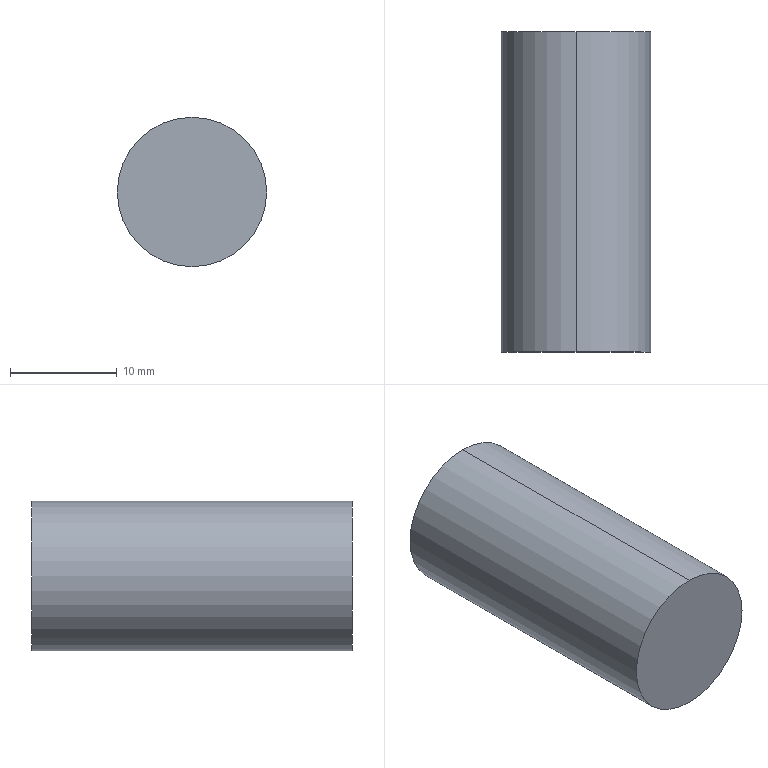Component | SolidWorks | DowelPin14X30-1 | 1 solid | 4 faces | box 14 x 30 x 14 mm | volume 4618 mm3 | cylinder 2 | plane 2 | commonest cylinder face diameters 14 x2
build123d program:
from build123d import *

# Parameters (mm, degrees)
SKETCH1_R           = 7
BOSS_EXTRUDE1_DEPTH = 30


with BuildPart() as part:
    # Sketch1 → Boss-Extrude1 (new body)
    with BuildSketch(Plane(origin=(0, 0, 0), x_dir=(1, 0, 0), z_dir=(0, 1, 0))):
        with Locations(Location((0, 0, 0), (0, 0, 270))):
            Circle(SKETCH1_R)
    extrude(amount=BOSS_EXTRUDE1_DEPTH)


solid = part.part

# Placed as in the assembly
solid = solid.moved(Location((-70.619, 73.047, -52), (0, 0, 0)))
STEP:
#1=COLOUR_RGB('',0.7922,0.8196,0.9333);
#2=FILL_AREA_STYLE_COLOUR('',#1);
#3=FILL_AREA_STYLE('',(#2));
#4=SURFACE_STYLE_FILL_AREA(#3);
#5=SURFACE_SIDE_STYLE('',(#4));
#6=SURFACE_STYLE_USAGE(.BOTH.,#5);
#7=PRESENTATION_STYLE_ASSIGNMENT((#6));
#8=CARTESIAN_POINT('',(-2.78,4.057,-1.772));
#9=VERTEX_POINT('',#8);
#10=CARTESIAN_POINT('',(-2.78,4.057,-2.323));
#11=VERTEX_POINT('',#10);
#12=CARTESIAN_POINT('',(-2.78,4.057,-2.047));
#13=DIRECTION('',(0.,1.,0.));
#14=DIRECTION('',(0.,0.,1.));
#15=AXIS2_PLACEMENT_3D('',#12,#13,#14);
#16=CIRCLE('',#15,0.2756);
#17=EDGE_CURVE('',#9,#11,#16,.T.);
#18=ORIENTED_EDGE('',*,*,#17,.F.);
#19=CARTESIAN_POINT('',(-2.78,2.876,-1.772));
#20=VERTEX_POINT('',#19);
#21=CARTESIAN_POINT('',(-2.78,4.057,-1.772));
#22=DIRECTION('',(0.,-1.,0.));
#23=VECTOR('',#22,39.37);
#24=LINE('',#21,#23);
#25=EDGE_CURVE('',#9,#20,#24,.T.);
#26=ORIENTED_EDGE('',*,*,#25,.T.);
#27=CARTESIAN_POINT('',(-2.78,2.876,-2.323));
#28=VERTEX_POINT('',#27);
#29=CARTESIAN_POINT('',(-2.78,2.876,-2.047));
#30=DIRECTION('',(0.,1.,0.));
#31=DIRECTION('',(0.,0.,1.));
#32=AXIS2_PLACEMENT_3D('',#29,#30,#31);
#33=CIRCLE('',#32,0.2756);
#34=EDGE_CURVE('',#20,#28,#33,.T.);
#35=ORIENTED_EDGE('',*,*,#34,.T.);
#36=CARTESIAN_POINT('',(-2.78,4.057,-2.323));
#37=DIRECTION('',(0.,-1.,0.));
#38=VECTOR('',#37,39.37);
#39=LINE('',#36,#38);
#40=EDGE_CURVE('',#11,#28,#39,.T.);
#41=ORIENTED_EDGE('',*,*,#40,.F.);
#42=EDGE_LOOP('',(#18,#26,#35,#41));
#43=FACE_OUTER_BOUND('',#42,.T.);
#44=CARTESIAN_POINT('',(-2.78,4.057,-2.047));
#45=DIRECTION('',(0.,-1.,0.));
#46=DIRECTION('',(0.,0.,-1.));
#47=AXIS2_PLACEMENT_3D('',#44,#45,#46);
#48=CYLINDRICAL_SURFACE('',#47,0.2756);
#49=ADVANCED_FACE('',(#43),#48,.T.);
#50=ORIENTED_EDGE('',*,*,#25,.F.);
#51=CARTESIAN_POINT('',(-2.78,4.057,-2.047));
#52=DIRECTION('',(0.,1.,0.));
#53=DIRECTION('',(0.,0.,1.));
#54=AXIS2_PLACEMENT_3D('',#51,#52,#53);
#55=CIRCLE('',#54,0.2756);
#56=EDGE_CURVE('',#11,#9,#55,.T.);
#57=ORIENTED_EDGE('',*,*,#56,.F.);
#58=ORIENTED_EDGE('',*,*,#40,.T.);
#59=CARTESIAN_POINT('',(-2.78,2.876,-2.047));
#60=DIRECTION('',(0.,1.,0.));
#61=DIRECTION('',(0.,0.,1.));
#62=AXIS2_PLACEMENT_3D('',#59,#60,#61);
#63=CIRCLE('',#62,0.2756);
#64=EDGE_CURVE('',#28,#20,#63,.T.);
#65=ORIENTED_EDGE('',*,*,#64,.T.);
#66=EDGE_LOOP('',(#50,#57,#58,#65));
#67=FACE_OUTER_BOUND('',#66,.T.);
#68=CARTESIAN_POINT('',(-2.78,4.057,-2.047));
#69=DIRECTION('',(0.,-1.,0.));
#70=DIRECTION('',(0.,0.,-1.));
#71=AXIS2_PLACEMENT_3D('',#68,#69,#70);
#72=CYLINDRICAL_SURFACE('',#71,0.2756);
#73=ADVANCED_FACE('',(#67),#72,.T.);
#74=ORIENTED_EDGE('',*,*,#56,.T.);
#75=ORIENTED_EDGE('',*,*,#17,.T.);
#76=EDGE_LOOP('',(#74,#75));
#77=FACE_OUTER_BOUND('',#76,.T.);
#78=CARTESIAN_POINT('',(-2.78,4.057,-2.047));
#79=DIRECTION('',(0.,1.,0.));
#80=DIRECTION('',(0.,0.,1.));
#81=AXIS2_PLACEMENT_3D('',#78,#79,#80);
#82=PLANE('',#81);
#83=ADVANCED_FACE('',(#77),#82,.T.);
#84=ORIENTED_EDGE('',*,*,#64,.F.);
#85=ORIENTED_EDGE('',*,*,#34,.F.);
#86=EDGE_LOOP('',(#84,#85));
#87=FACE_OUTER_BOUND('',#86,.T.);
#88=CARTESIAN_POINT('',(-2.78,2.876,-2.047));
#89=DIRECTION('',(0.,1.,0.));
#90=DIRECTION('',(0.,0.,1.));
#91=AXIS2_PLACEMENT_3D('',#88,#89,#90);
#92=PLANE('',#91);
#93=ADVANCED_FACE('',(#87),#92,.F.);
#94=CLOSED_SHELL('',(#49,#73,#83,#93));
#95=MANIFOLD_SOLID_BREP('',#94);
#96=STYLED_ITEM('',(#7),#95);
#97=PRESENTATION_LAYER_ASSIGNMENT('','',(#96));
#98=CARTESIAN_POINT('',(0.,0.,0.));
#99=DIRECTION('',(0.,0.,1.));
#100=DIRECTION('',(1.,0.,0.));
#101=AXIS2_PLACEMENT_3D('',#98,#99,#100);
#102=(LENGTH_UNIT()NAMED_UNIT(*)SI_UNIT($,.METRE.));
#103=LENGTH_MEASURE_WITH_UNIT(LENGTH_MEASURE(0.0254),#102);
#104=DIMENSIONAL_EXPONENTS(1.,0.,0.,0.,0.,0.,0.);
#105=(CONVERSION_BASED_UNIT('',#103)LENGTH_UNIT()NAMED_UNIT(#104));
#106=UNCERTAINTY_MEASURE_WITH_UNIT(LENGTH_MEASURE(0.00001),#105,'','');
#107=(NAMED_UNIT(*)PLANE_ANGLE_UNIT()SI_UNIT($,.RADIAN.));
#108=(NAMED_UNIT(*)SI_UNIT($,.STERADIAN.)SOLID_ANGLE_UNIT());
#109=(GEOMETRIC_REPRESENTATION_CONTEXT(3)GLOBAL_UNCERTAINTY_ASSIGNED_CONTEXT((#106))GLOBAL_UNIT_ASSIGNED_CONTEXT((#105,#107,#108))REPRESENTATION_CONTEXT('',''));
#110=ADVANCED_BREP_SHAPE_REPRESENTATION('',(#95,#101),#109);
#111=(LENGTH_UNIT()NAMED_UNIT(*)SI_UNIT($,.METRE.));
#112=LENGTH_MEASURE_WITH_UNIT(LENGTH_MEASURE(0.0254),#111);
#113=DIMENSIONAL_EXPONENTS(1.,0.,0.,0.,0.,0.,0.);
#114=(CONVERSION_BASED_UNIT('',#112)LENGTH_UNIT()NAMED_UNIT(#113));
#115=UNCERTAINTY_MEASURE_WITH_UNIT(LENGTH_MEASURE(0.00001),#114,'','');
#116=(NAMED_UNIT(*)PLANE_ANGLE_UNIT()SI_UNIT($,.RADIAN.));
#117=(NAMED_UNIT(*)SI_UNIT($,.STERADIAN.)SOLID_ANGLE_UNIT());
#118=(GEOMETRIC_REPRESENTATION_CONTEXT(3)GLOBAL_UNCERTAINTY_ASSIGNED_CONTEXT((#115))GLOBAL_UNIT_ASSIGNED_CONTEXT((#114,#116,#117))REPRESENTATION_CONTEXT('',''));
#119=MECHANICAL_DESIGN_GEOMETRIC_PRESENTATION_REPRESENTATION('',(#96),#118);